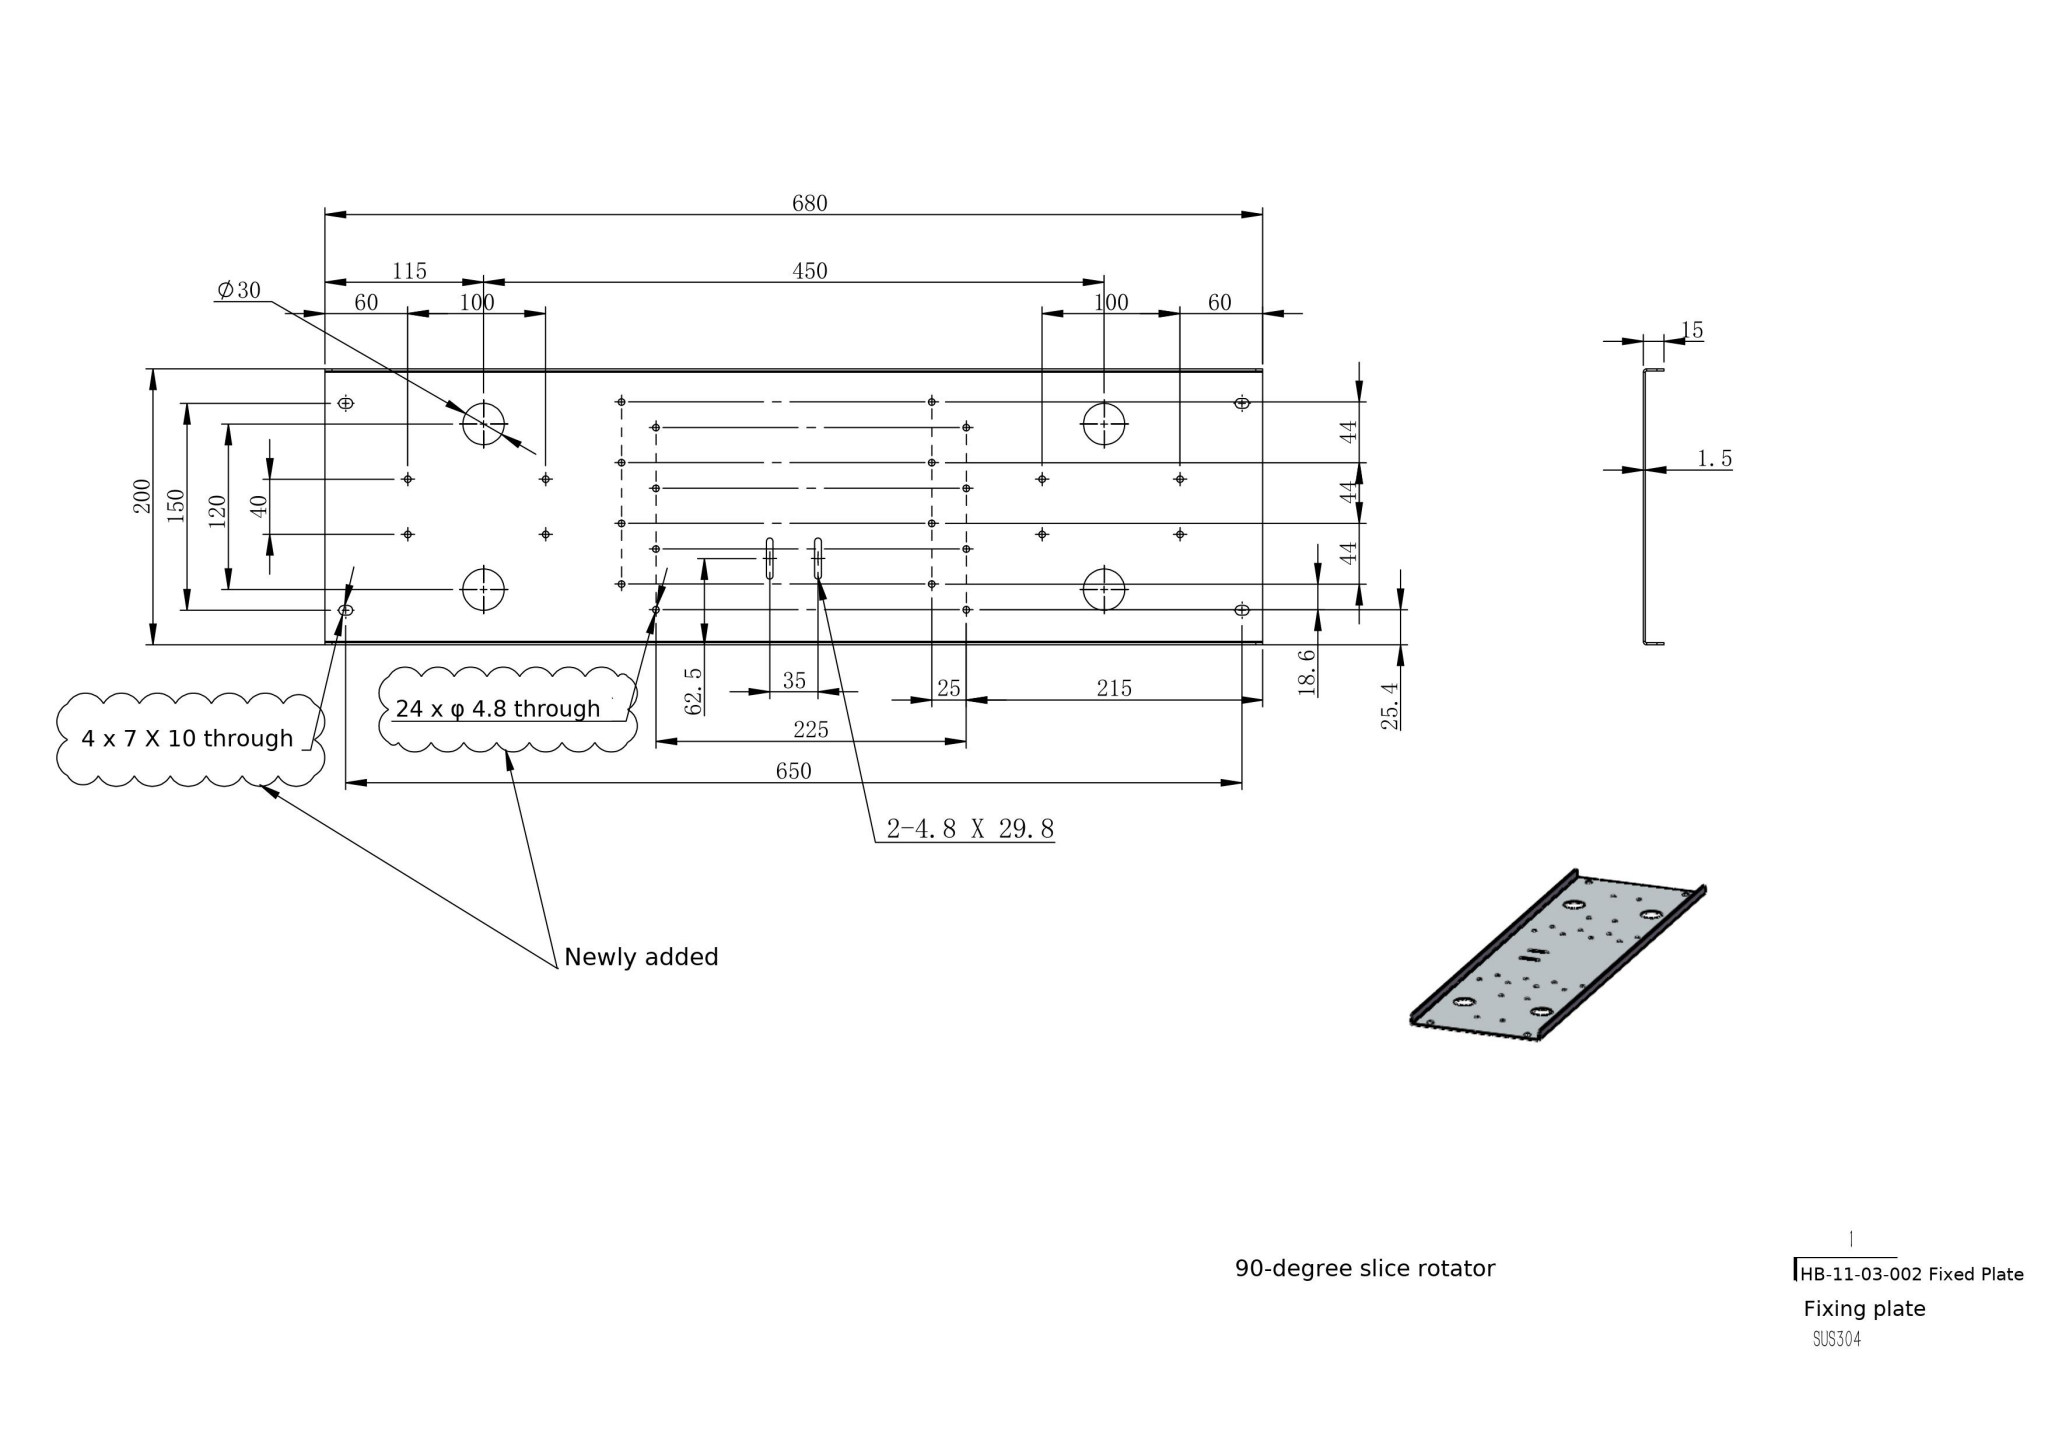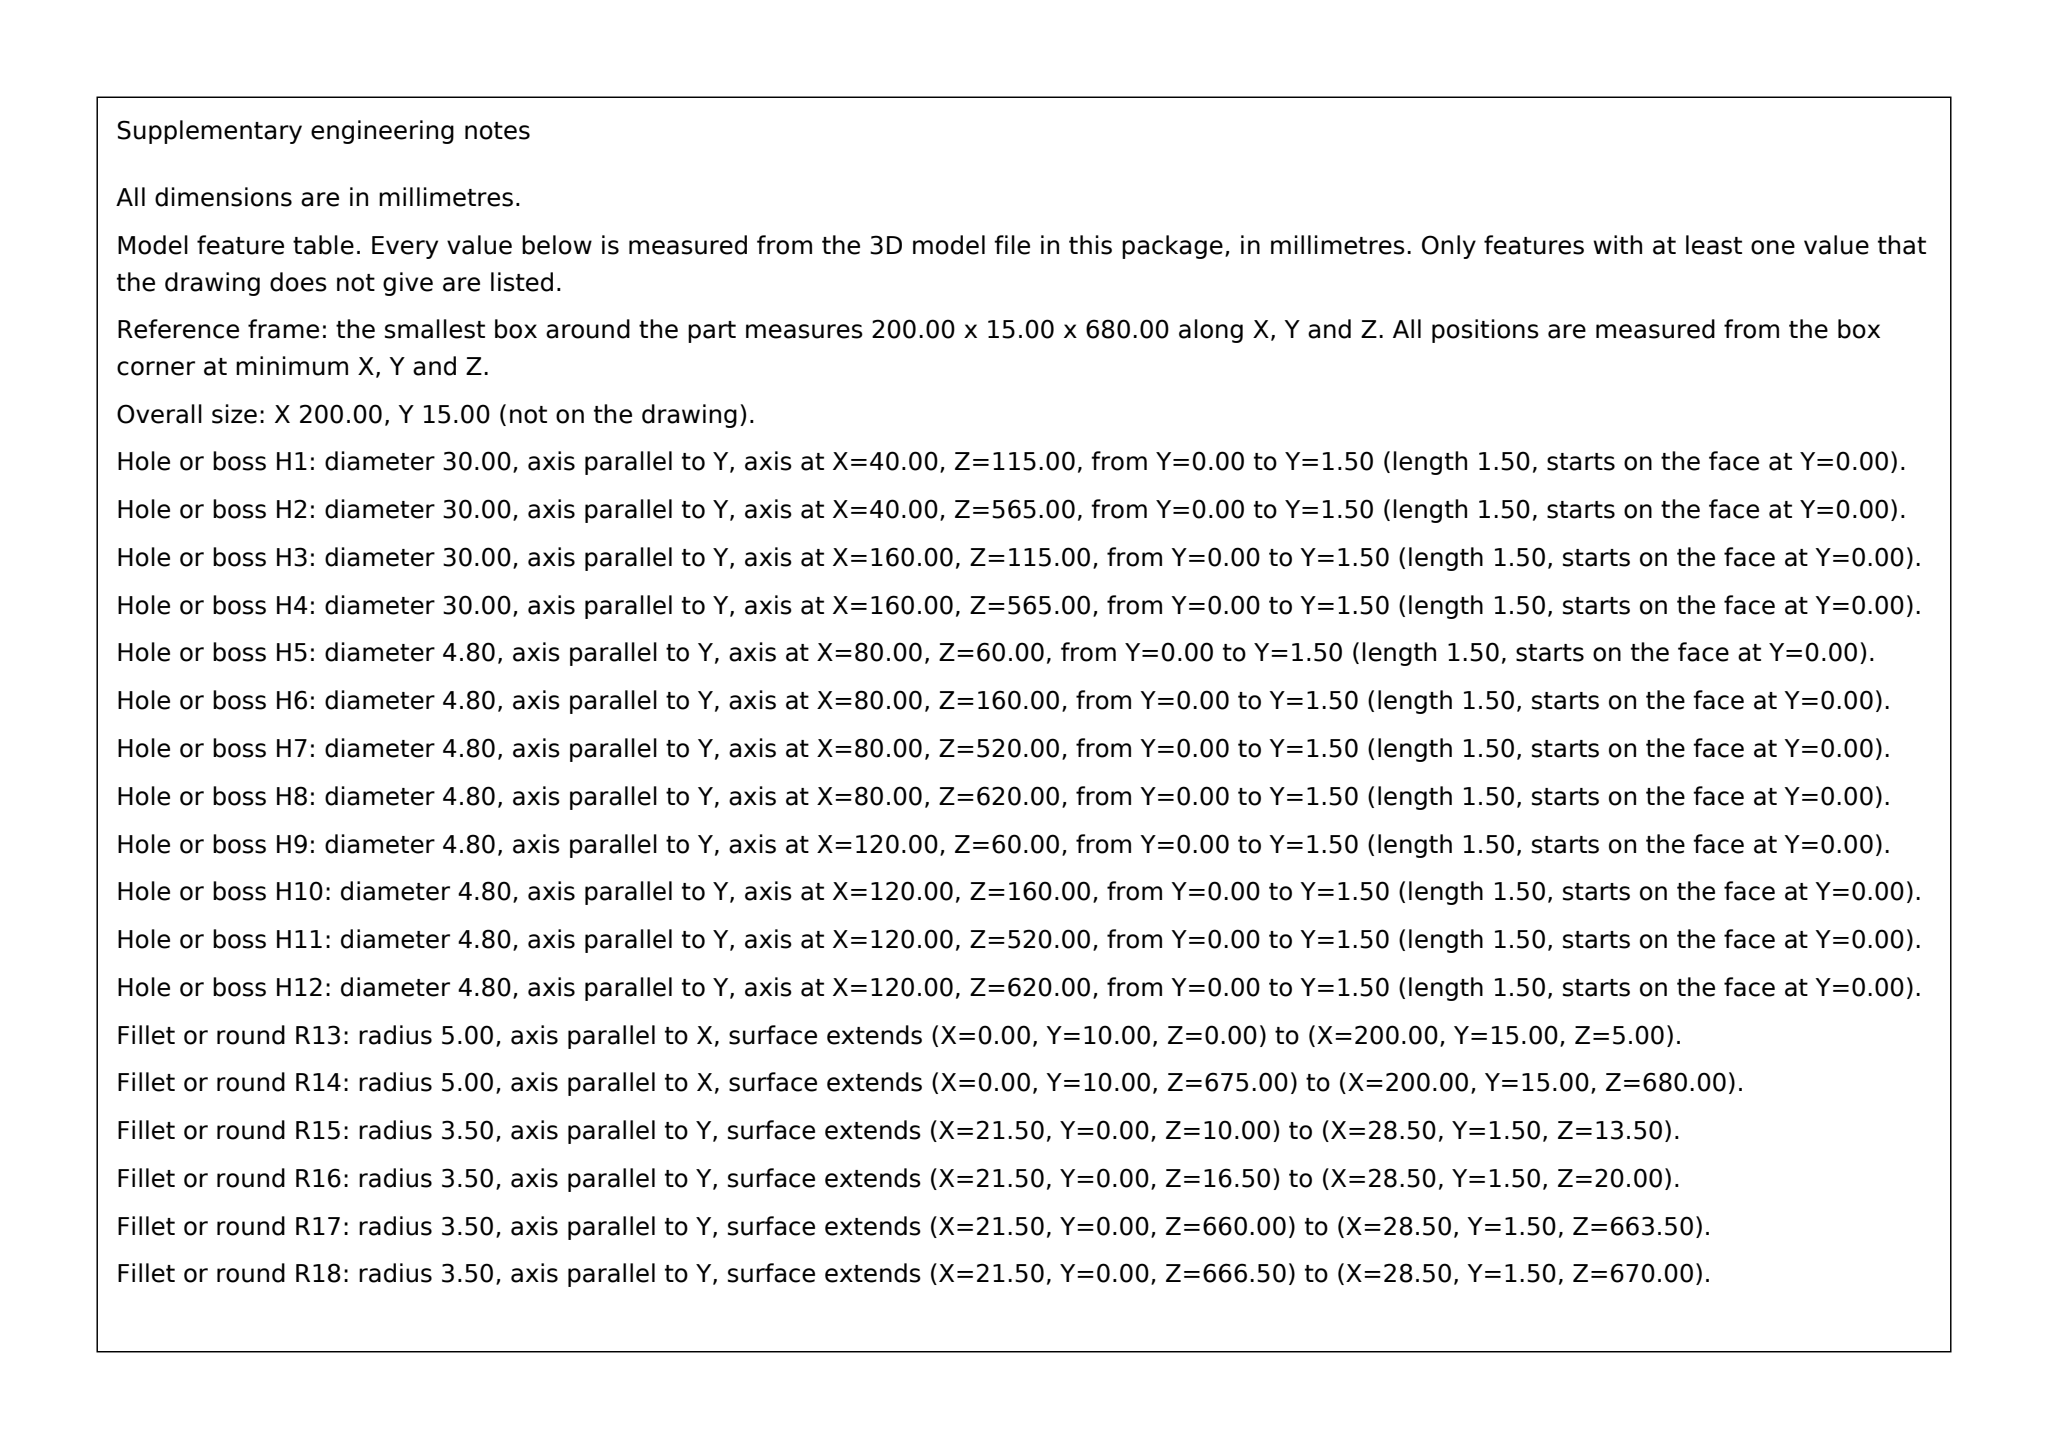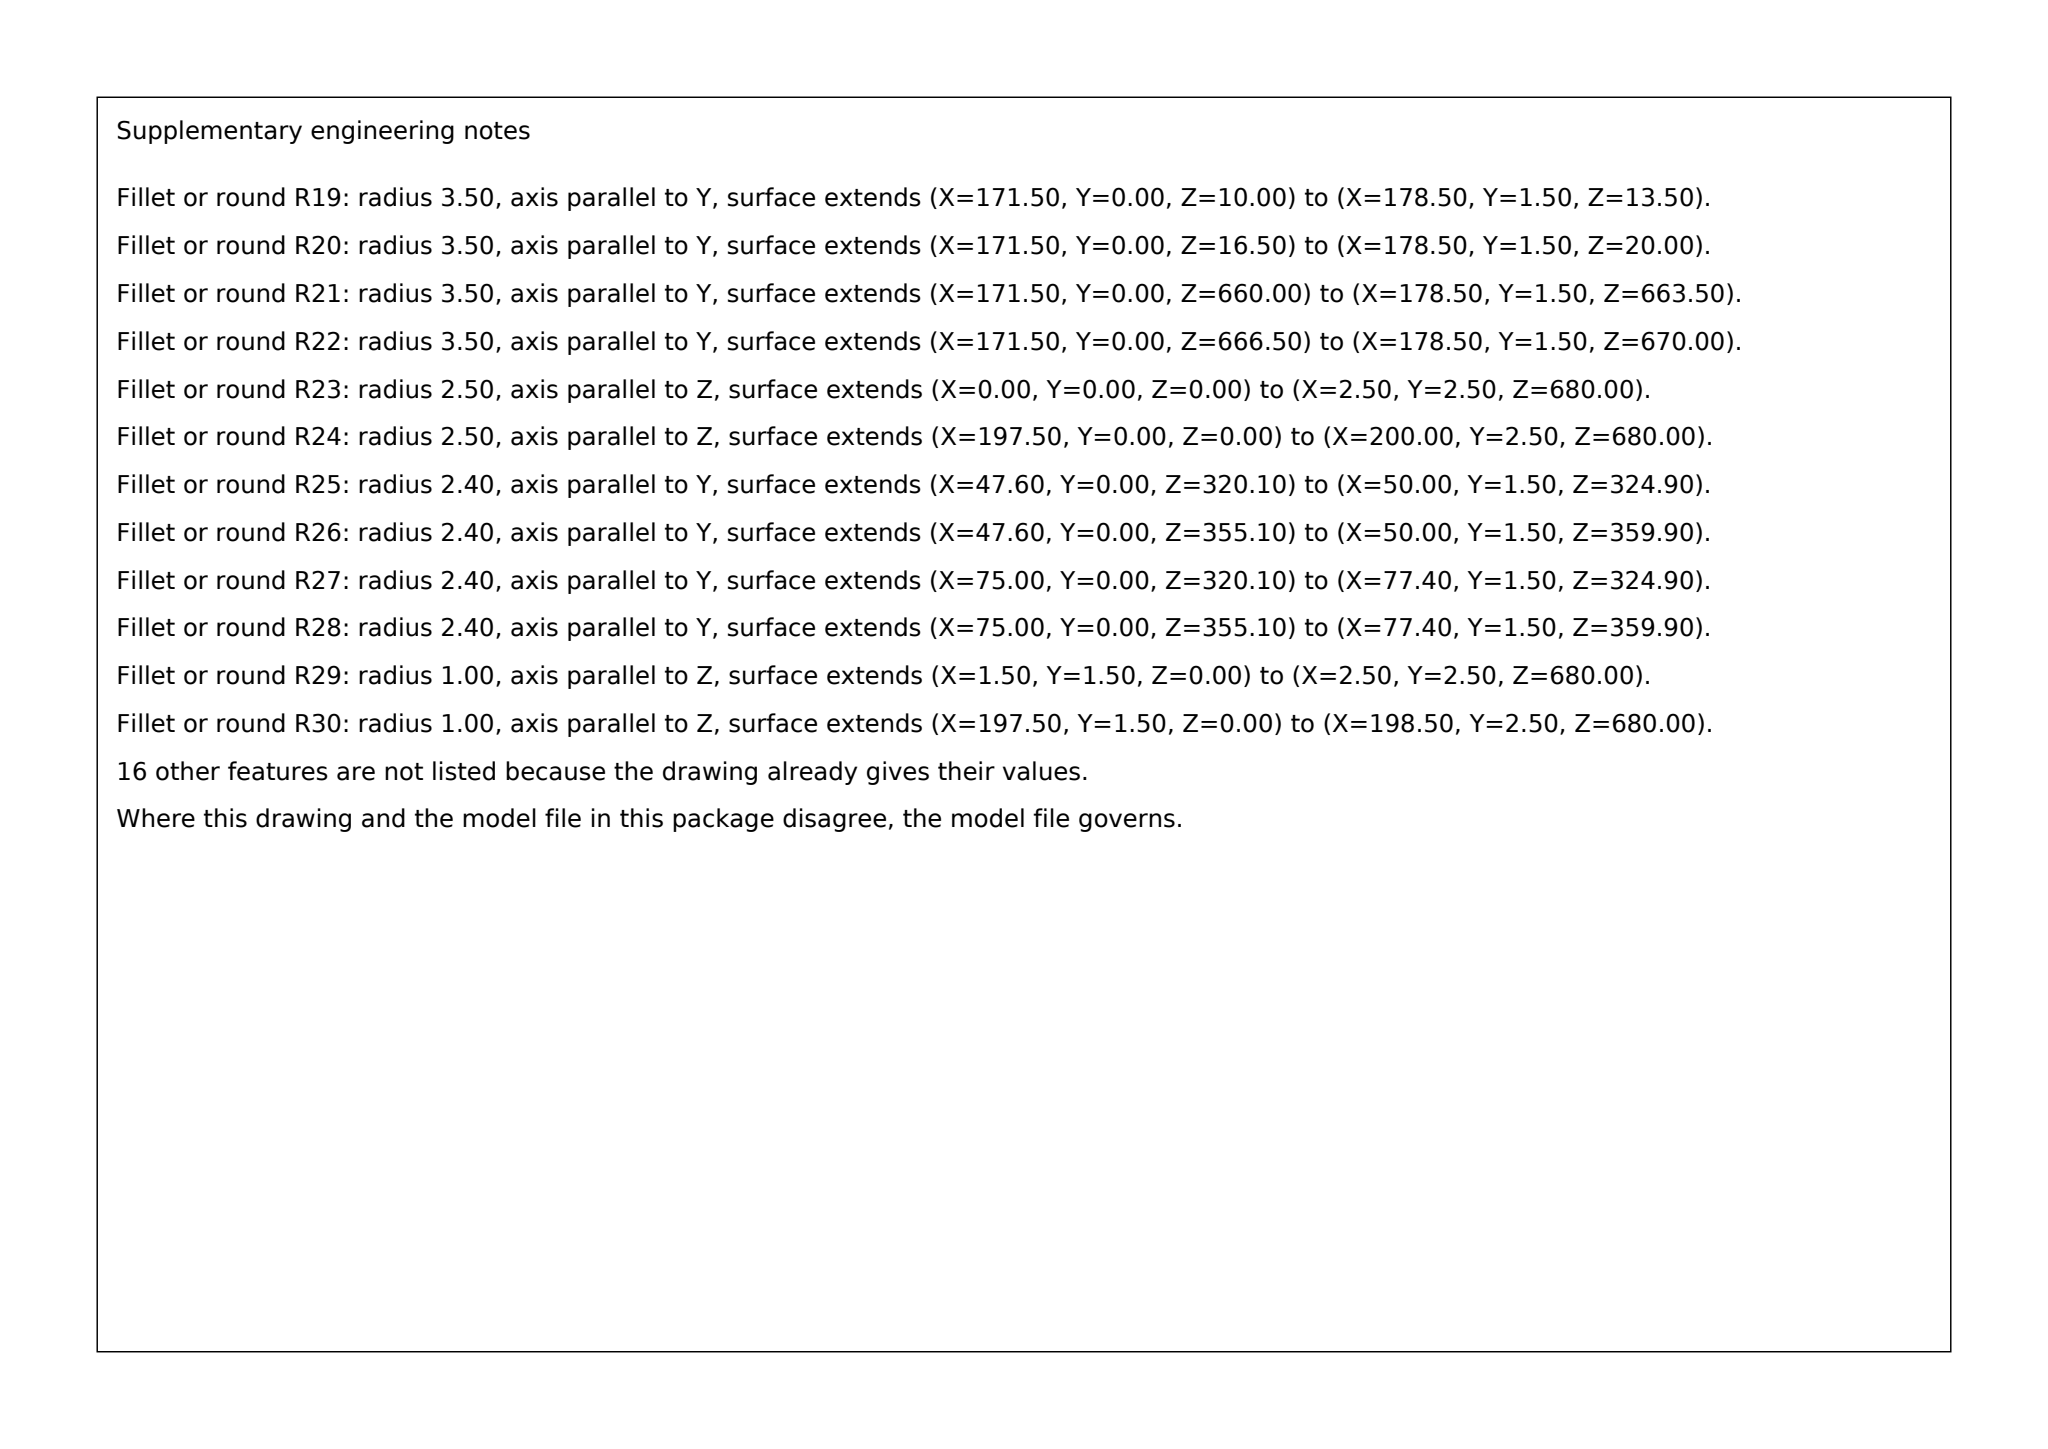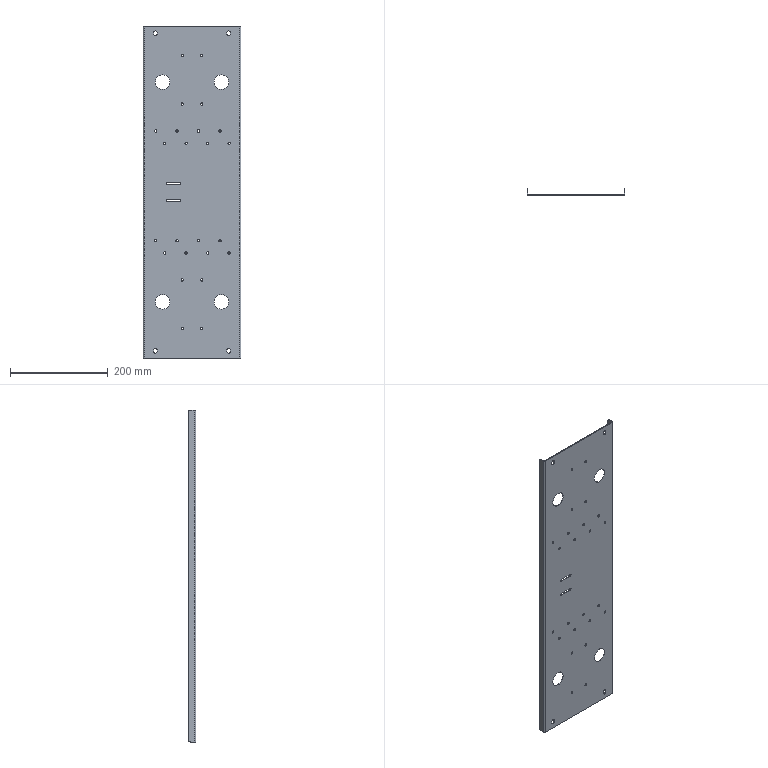Part | SolidWorks | mm | material SUS304 | 1 solid | 110 faces | box 200 x 15 x 680 mm | volume 224312 mm3 | cylinder 80 | plane 30 | commonest cylinder face diameters 4.8 x52 7 x12 30 x8 10 x4 5 x2 2 x2